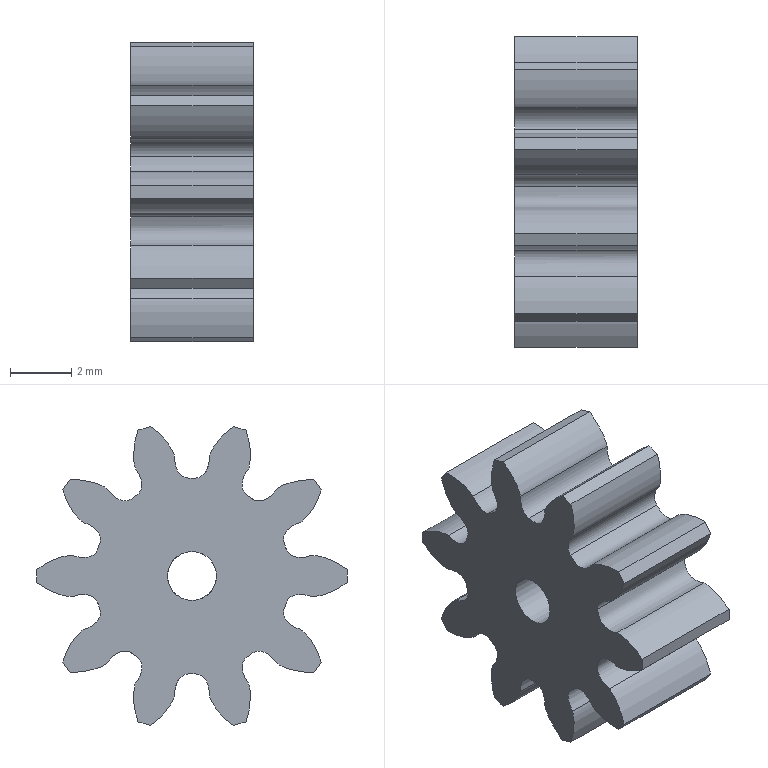Component | NX | GEAR_2_2 | 1 solid | 53 faces | volume 206 mm3 | spline 50 | plane 2 | cylinder 1 | commonest cylinder face diameters 1.6 x1